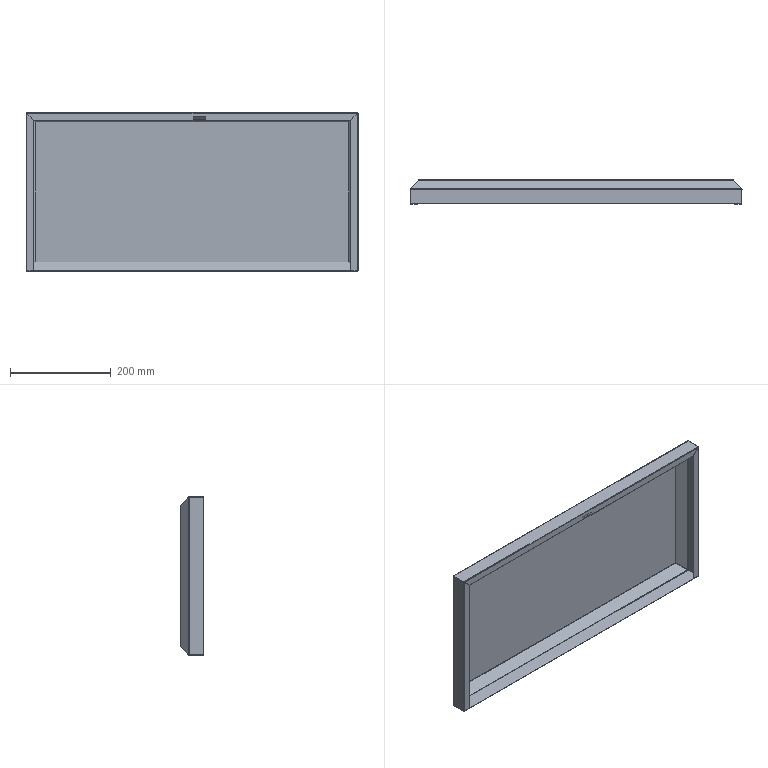Component | SolidWorks | PC-CAJ-P09-1_PM-CAJ-P50-1 | 1 solid | 106 faces | volume 206839 mm3 | plane 72 | cylinder 22 | spline 12 | commonest cylinder face diameters 1 x11 2.4 x11 | material Plain Carbon Steel